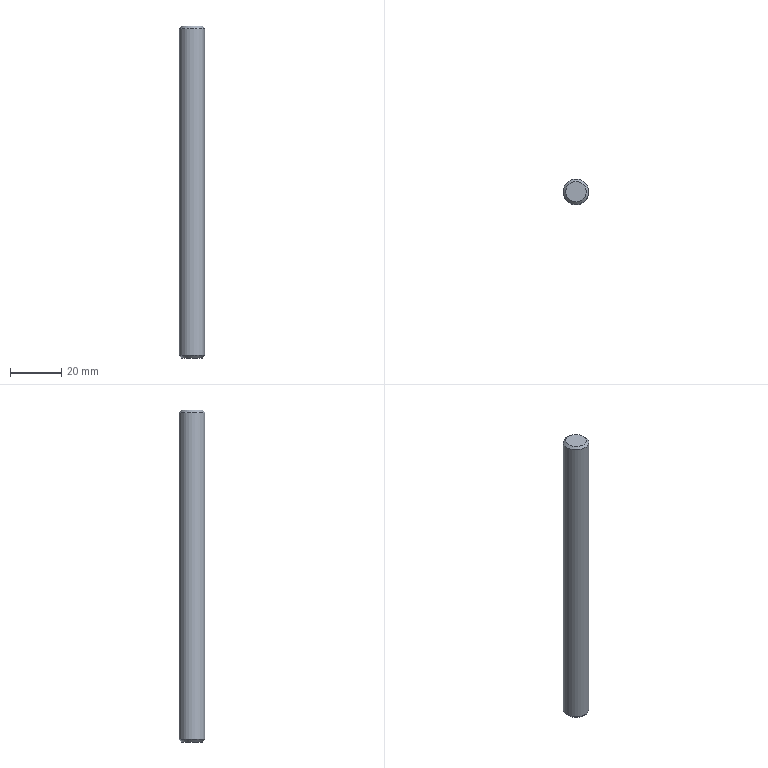Component | NX | DOWEL_PIN_130_3 | 1 solid | 5 faces | box 10 x 10 x 130 mm | volume 10181 mm3 | plane 2 | cone 2 | cylinder 1 | commonest cylinder face diameters 10 x1
STEP:
#1=CARTESIAN_POINT('',(0.,0.,0.));
#2=DIRECTION('',(0.,0.,1.));
#3=DIRECTION('',(1.,0.,0.));
#4=AXIS2_PLACEMENT_3D('',#1,#2,#3);
#5=CARTESIAN_POINT('',(204.,120.,240.));
#6=VERTEX_POINT('',#5);
#7=CARTESIAN_POINT('',(200.,120.,240.));
#8=DIRECTION('',(0.,0.,1.));
#9=DIRECTION('',(1.,0.,0.));
#10=AXIS2_PLACEMENT_3D('',#7,#8,#9);
#11=CIRCLE('',#10,4.);
#12=CARTESIAN_POINT('',(200.,120.,240.));
#13=DIRECTION('',(0.,0.,1.));
#14=DIRECTION('',(1.,0.,0.));
#15=AXIS2_PLACEMENT_3D('',#12,#13,#14);
#16=PLANE('',#15);
#17=CARTESIAN_POINT('',(0.,0.));
#18=DIRECTION('',(1.,0.));
#19=AXIS2_PLACEMENT_2D('',#17,#18);
#20=CIRCLE('',#19,4.);
#21=(GEOMETRIC_REPRESENTATION_CONTEXT(2)PARAMETRIC_REPRESENTATION_CONTEXT()REPRESENTATION_CONTEXT('',''));
#22=DEFINITIONAL_REPRESENTATION('',(#20),#21);
#23=PCURVE('',#16,#22);
#24=CARTESIAN_POINT('',(200.,120.,239.));
#25=DIRECTION('',(0.,0.,-1.));
#26=DIRECTION('',(-1.,0.,0.));
#27=AXIS2_PLACEMENT_3D('',#24,#25,#26);
#28=CONICAL_SURFACE('',#27,5.,0.7854);
#29=CARTESIAN_POINT('',(9.425,-1.));
#30=DIRECTION('',(-1.,0.));
#31=VECTOR('',#30,1.);
#32=LINE('',#29,#31);
#33=(GEOMETRIC_REPRESENTATION_CONTEXT(2)PARAMETRIC_REPRESENTATION_CONTEXT()REPRESENTATION_CONTEXT('',''));
#34=DEFINITIONAL_REPRESENTATION('',(#32),#33);
#35=PCURVE('',#28,#34);
#36=SURFACE_CURVE('',#11,(#23,#35),.PCURVE_S1.);
#37=EDGE_CURVE('',#6,#6,#36,.T.);
#38=ORIENTED_EDGE('',*,*,#37,.T.);
#39=EDGE_LOOP('',(#38));
#40=FACE_BOUND('',#39,.T.);
#41=ADVANCED_FACE('',(#40),#16,.T.);
#42=CARTESIAN_POINT('',(196.,120.,110.));
#43=VERTEX_POINT('',#42);
#44=CARTESIAN_POINT('',(200.,120.,110.));
#45=DIRECTION('',(0.,0.,-1.));
#46=DIRECTION('',(-1.,0.,0.));
#47=AXIS2_PLACEMENT_3D('',#44,#45,#46);
#48=CIRCLE('',#47,4.);
#49=CARTESIAN_POINT('',(200.,120.,110.));
#50=DIRECTION('',(0.,0.,-1.));
#51=DIRECTION('',(-1.,0.,0.));
#52=AXIS2_PLACEMENT_3D('',#49,#50,#51);
#53=PLANE('',#52);
#54=CARTESIAN_POINT('',(0.,0.));
#55=DIRECTION('',(1.,0.));
#56=AXIS2_PLACEMENT_2D('',#54,#55);
#57=CIRCLE('',#56,4.);
#58=(GEOMETRIC_REPRESENTATION_CONTEXT(2)PARAMETRIC_REPRESENTATION_CONTEXT()REPRESENTATION_CONTEXT('',''));
#59=DEFINITIONAL_REPRESENTATION('',(#57),#58);
#60=PCURVE('',#53,#59);
#61=CARTESIAN_POINT('',(200.,120.,111.));
#62=DIRECTION('',(0.,0.,1.));
#63=DIRECTION('',(1.,0.,0.));
#64=AXIS2_PLACEMENT_3D('',#61,#62,#63);
#65=CONICAL_SURFACE('',#64,5.,0.7854);
#66=CARTESIAN_POINT('',(9.425,-1.));
#67=DIRECTION('',(-1.,0.));
#68=VECTOR('',#67,1.);
#69=LINE('',#66,#68);
#70=(GEOMETRIC_REPRESENTATION_CONTEXT(2)PARAMETRIC_REPRESENTATION_CONTEXT()REPRESENTATION_CONTEXT('',''));
#71=DEFINITIONAL_REPRESENTATION('',(#69),#70);
#72=PCURVE('',#65,#71);
#73=SURFACE_CURVE('',#48,(#60,#72),.PCURVE_S1.);
#74=EDGE_CURVE('',#43,#43,#73,.T.);
#75=ORIENTED_EDGE('',*,*,#74,.T.);
#76=EDGE_LOOP('',(#75));
#77=FACE_BOUND('',#76,.T.);
#78=ADVANCED_FACE('',(#77),#53,.T.);
#79=CARTESIAN_POINT('',(195.,120.,111.));
#80=VERTEX_POINT('',#79);
#81=CARTESIAN_POINT('',(205.,120.,111.));
#82=VERTEX_POINT('',#81);
#83=CARTESIAN_POINT('',(200.,120.,111.));
#84=DIRECTION('',(0.,0.,1.));
#85=DIRECTION('',(-1.,0.,0.));
#86=AXIS2_PLACEMENT_3D('',#83,#84,#85);
#87=CIRCLE('',#86,5.);
#88=CARTESIAN_POINT('',(200.,120.,110.));
#89=DIRECTION('',(0.,0.,1.));
#90=DIRECTION('',(1.,0.,0.));
#91=AXIS2_PLACEMENT_3D('',#88,#89,#90);
#92=CYLINDRICAL_SURFACE('',#91,5.);
#93=CARTESIAN_POINT('',(3.142,1.));
#94=DIRECTION('',(1.,0.));
#95=VECTOR('',#94,1.);
#96=LINE('',#93,#95);
#97=(GEOMETRIC_REPRESENTATION_CONTEXT(2)PARAMETRIC_REPRESENTATION_CONTEXT()REPRESENTATION_CONTEXT('',''));
#98=DEFINITIONAL_REPRESENTATION('',(#96),#97);
#99=PCURVE('',#92,#98);
#100=CARTESIAN_POINT('',(3.142,0.));
#101=DIRECTION('',(1.,0.));
#102=VECTOR('',#101,1.);
#103=LINE('',#100,#102);
#104=(GEOMETRIC_REPRESENTATION_CONTEXT(2)PARAMETRIC_REPRESENTATION_CONTEXT()REPRESENTATION_CONTEXT('',''));
#105=DEFINITIONAL_REPRESENTATION('',(#103),#104);
#106=PCURVE('',#65,#105);
#107=SURFACE_CURVE('',#87,(#99,#106),.PCURVE_S1.);
#108=EDGE_CURVE('',#80,#82,#107,.T.);
#109=ORIENTED_EDGE('',*,*,#108,.T.);
#110=CARTESIAN_POINT('',(205.,120.,239.));
#111=VERTEX_POINT('',#110);
#112=CARTESIAN_POINT('',(205.,120.,111.));
#113=CARTESIAN_POINT('',(205.,120.,239.));
#114=B_SPLINE_CURVE_WITH_KNOTS('',1,(#112,#113),.UNSPECIFIED.,.F.,.F.,(2,2),(1.,129.),.PIECEWISE_BEZIER_KNOTS.);
#115=CARTESIAN_POINT('',(6.283,0.));
#116=DIRECTION('',(0.,1.));
#117=VECTOR('',#116,1.);
#118=LINE('',#115,#117);
#119=(GEOMETRIC_REPRESENTATION_CONTEXT(2)PARAMETRIC_REPRESENTATION_CONTEXT()REPRESENTATION_CONTEXT('',''));
#120=DEFINITIONAL_REPRESENTATION('',(#118),#119);
#121=PCURVE('',#92,#120);
#122=CARTESIAN_POINT('',(0.,0.));
#123=DIRECTION('',(0.,1.));
#124=VECTOR('',#123,1.);
#125=LINE('',#122,#124);
#126=(GEOMETRIC_REPRESENTATION_CONTEXT(2)PARAMETRIC_REPRESENTATION_CONTEXT()REPRESENTATION_CONTEXT('',''));
#127=DEFINITIONAL_REPRESENTATION('',(#125),#126);
#128=PCURVE('',#92,#127);
#129=SEAM_CURVE('',#114,(#121,#128),.PCURVE_S1.);
#130=EDGE_CURVE('',#82,#111,#129,.T.);
#131=ORIENTED_EDGE('',*,*,#130,.T.);
#132=CARTESIAN_POINT('',(200.,120.,239.));
#133=DIRECTION('',(0.,0.,-1.));
#134=DIRECTION('',(1.,0.,0.));
#135=AXIS2_PLACEMENT_3D('',#132,#133,#134);
#136=CIRCLE('',#135,5.);
#137=CARTESIAN_POINT('',(6.283,129.));
#138=DIRECTION('',(-1.,0.));
#139=VECTOR('',#138,1.);
#140=LINE('',#137,#139);
#141=(GEOMETRIC_REPRESENTATION_CONTEXT(2)PARAMETRIC_REPRESENTATION_CONTEXT()REPRESENTATION_CONTEXT('',''));
#142=DEFINITIONAL_REPRESENTATION('',(#140),#141);
#143=PCURVE('',#92,#142);
#144=CARTESIAN_POINT('',(3.142,0.));
#145=DIRECTION('',(1.,0.));
#146=VECTOR('',#145,1.);
#147=LINE('',#144,#146);
#148=(GEOMETRIC_REPRESENTATION_CONTEXT(2)PARAMETRIC_REPRESENTATION_CONTEXT()REPRESENTATION_CONTEXT('',''));
#149=DEFINITIONAL_REPRESENTATION('',(#147),#148);
#150=PCURVE('',#28,#149);
#151=SURFACE_CURVE('',#136,(#143,#150),.PCURVE_S1.);
#152=EDGE_CURVE('',#111,#111,#151,.T.);
#153=ORIENTED_EDGE('',*,*,#152,.T.);
#154=ORIENTED_EDGE('',*,*,#130,.F.);
#155=CARTESIAN_POINT('',(200.,120.,111.));
#156=DIRECTION('',(0.,0.,1.));
#157=DIRECTION('',(-1.,0.,0.));
#158=AXIS2_PLACEMENT_3D('',#155,#156,#157);
#159=CIRCLE('',#158,5.);
#160=CARTESIAN_POINT('',(-3.142,1.));
#161=DIRECTION('',(1.,0.));
#162=VECTOR('',#161,1.);
#163=LINE('',#160,#162);
#164=(GEOMETRIC_REPRESENTATION_CONTEXT(2)PARAMETRIC_REPRESENTATION_CONTEXT()REPRESENTATION_CONTEXT('',''));
#165=DEFINITIONAL_REPRESENTATION('',(#163),#164);
#166=PCURVE('',#92,#165);
#167=CARTESIAN_POINT('',(3.142,0.));
#168=DIRECTION('',(1.,0.));
#169=VECTOR('',#168,1.);
#170=LINE('',#167,#169);
#171=(GEOMETRIC_REPRESENTATION_CONTEXT(2)PARAMETRIC_REPRESENTATION_CONTEXT()REPRESENTATION_CONTEXT('',''));
#172=DEFINITIONAL_REPRESENTATION('',(#170),#171);
#173=PCURVE('',#65,#172);
#174=SURFACE_CURVE('',#159,(#166,#173),.PCURVE_S1.);
#175=EDGE_CURVE('',#82,#80,#174,.T.);
#176=ORIENTED_EDGE('',*,*,#175,.T.);
#177=EDGE_LOOP('',(#109,#131,#153,#154,#176));
#178=FACE_BOUND('',#177,.T.);
#179=ADVANCED_FACE('',(#178),#92,.T.);
#180=ORIENTED_EDGE('',*,*,#74,.F.);
#181=CARTESIAN_POINT('',(196.,120.,110.));
#182=CARTESIAN_POINT('',(195.,120.,111.));
#183=B_SPLINE_CURVE_WITH_KNOTS('',1,(#181,#182),.UNSPECIFIED.,.F.,.F.,(2,2),(-1.414,0.),.PIECEWISE_BEZIER_KNOTS.);
#184=CARTESIAN_POINT('',(9.425,0.));
#185=DIRECTION('',(0.,1.));
#186=VECTOR('',#185,1.);
#187=LINE('',#184,#186);
#188=(GEOMETRIC_REPRESENTATION_CONTEXT(2)PARAMETRIC_REPRESENTATION_CONTEXT()REPRESENTATION_CONTEXT('',''));
#189=DEFINITIONAL_REPRESENTATION('',(#187),#188);
#190=PCURVE('',#65,#189);
#191=CARTESIAN_POINT('',(3.142,0.));
#192=DIRECTION('',(0.,1.));
#193=VECTOR('',#192,1.);
#194=LINE('',#191,#193);
#195=(GEOMETRIC_REPRESENTATION_CONTEXT(2)PARAMETRIC_REPRESENTATION_CONTEXT()REPRESENTATION_CONTEXT('',''));
#196=DEFINITIONAL_REPRESENTATION('',(#194),#195);
#197=PCURVE('',#65,#196);
#198=SEAM_CURVE('',#183,(#190,#197),.PCURVE_S1.);
#199=EDGE_CURVE('',#43,#80,#198,.T.);
#200=ORIENTED_EDGE('',*,*,#199,.T.);
#201=ORIENTED_EDGE('',*,*,#175,.F.);
#202=ORIENTED_EDGE('',*,*,#108,.F.);
#203=ORIENTED_EDGE('',*,*,#199,.F.);
#204=EDGE_LOOP('',(#180,#200,#201,#202,#203));
#205=FACE_BOUND('',#204,.T.);
#206=ADVANCED_FACE('',(#205),#65,.T.);
#207=ORIENTED_EDGE('',*,*,#37,.F.);
#208=CARTESIAN_POINT('',(204.,120.,240.));
#209=CARTESIAN_POINT('',(205.,120.,239.));
#210=B_SPLINE_CURVE_WITH_KNOTS('',1,(#208,#209),.UNSPECIFIED.,.F.,.F.,(2,2),(-1.414,0.),.PIECEWISE_BEZIER_KNOTS.);
#211=CARTESIAN_POINT('',(9.425,0.));
#212=DIRECTION('',(0.,1.));
#213=VECTOR('',#212,1.);
#214=LINE('',#211,#213);
#215=(GEOMETRIC_REPRESENTATION_CONTEXT(2)PARAMETRIC_REPRESENTATION_CONTEXT()REPRESENTATION_CONTEXT('',''));
#216=DEFINITIONAL_REPRESENTATION('',(#214),#215);
#217=PCURVE('',#28,#216);
#218=CARTESIAN_POINT('',(3.142,0.));
#219=DIRECTION('',(0.,1.));
#220=VECTOR('',#219,1.);
#221=LINE('',#218,#220);
#222=(GEOMETRIC_REPRESENTATION_CONTEXT(2)PARAMETRIC_REPRESENTATION_CONTEXT()REPRESENTATION_CONTEXT('',''));
#223=DEFINITIONAL_REPRESENTATION('',(#221),#222);
#224=PCURVE('',#28,#223);
#225=SEAM_CURVE('',#210,(#217,#224),.PCURVE_S1.);
#226=EDGE_CURVE('',#6,#111,#225,.T.);
#227=ORIENTED_EDGE('',*,*,#226,.T.);
#228=ORIENTED_EDGE('',*,*,#152,.F.);
#229=ORIENTED_EDGE('',*,*,#226,.F.);
#230=EDGE_LOOP('',(#207,#227,#228,#229));
#231=FACE_BOUND('',#230,.T.);
#232=ADVANCED_FACE('',(#231),#28,.T.);
#233=CLOSED_SHELL('',(#41,#78,#179,#206,#232));
#234=MANIFOLD_SOLID_BREP('',#233);
#235=(LENGTH_UNIT()NAMED_UNIT(*)SI_UNIT(.MILLI.,.METRE.));
#236=UNCERTAINTY_MEASURE_WITH_UNIT(LENGTH_MEASURE(0.00001),#235,'','');
#237=(NAMED_UNIT(*)PLANE_ANGLE_UNIT()SI_UNIT($,.RADIAN.));
#238=(NAMED_UNIT(*)SI_UNIT($,.STERADIAN.)SOLID_ANGLE_UNIT());
#239=(GEOMETRIC_REPRESENTATION_CONTEXT(3)GLOBAL_UNCERTAINTY_ASSIGNED_CONTEXT((#236))GLOBAL_UNIT_ASSIGNED_CONTEXT((#235,#237,#238))REPRESENTATION_CONTEXT('',''));
#240=ADVANCED_BREP_SHAPE_REPRESENTATION('',(#4,#234),#239);